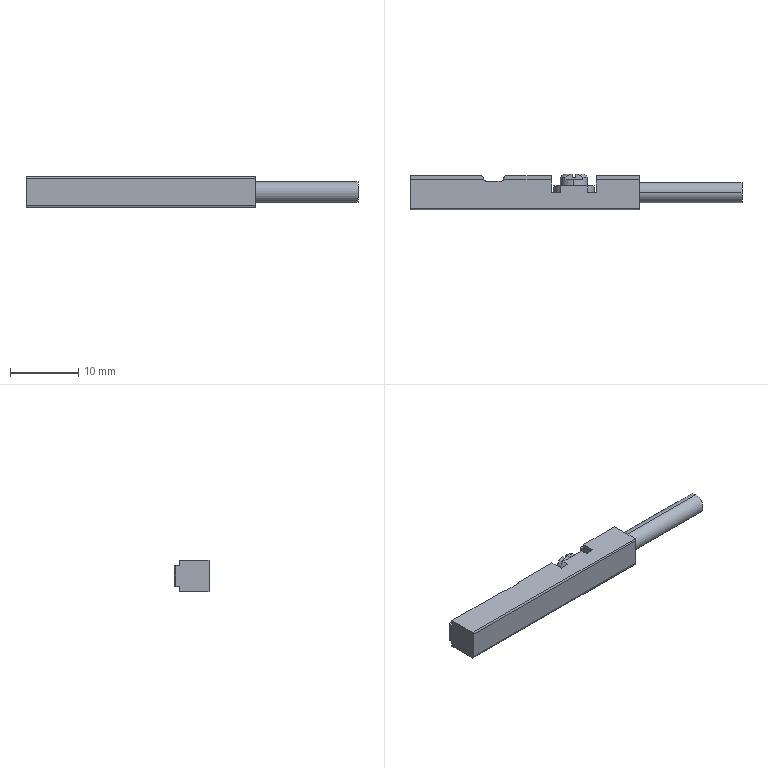Component | SolidWorks | BearingLiftingModule-1_RMT16X100S_0_+_CS1-G-2-1_CS1-E-1 | 1 solid | 50 faces | volume 816 mm3 | plane 36 | cylinder 12 | cone 2 | commonest cylinder face diameters 0.8 x4 3 x2 4 x2 6 x2 1 x2